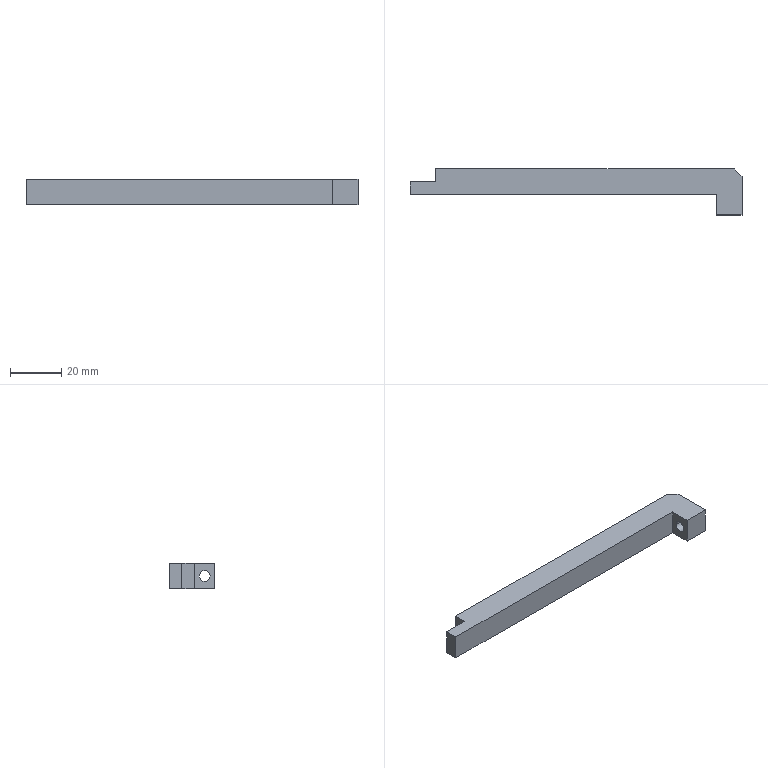Component | SolidWorks | SecondGenerationFour-sidedLabelingFeedingFrontLimitPlate-1 | 1 solid | 13 faces | box 130 x 18 x 10 mm | volume 13116 mm3 | plane 11 | cylinder 2 | commonest cylinder face diameters 4.2 x2
build123d program:
from build123d import *

# Parameters (mm, degrees)
SKETCH1_W             = 120
SKETCH1_H             = 10
BOSS_EXTRUDE1_DEPTH   = 10
SKETCH2_W             = 10
SKETCH2_H             = 10
BOSS_EXTRUDE2_DEPTH   = 8
M5_TAPPED_HOLE1_D     = 4.2
M5_TAPPED_HOLE1_DEPTH = 19
M5_TAPPED_HOLE1_TIP   = 1.262
SKETCH6_W             = 5
SKETCH6_H             = 10
BOSS_EXTRUDE4_DEPTH   = 10
CHAMFER1_SIZE         = 3


with BuildPart() as part:
    # Sketch1 → Boss-Extrude1 (new body)
    with BuildSketch(Plane.XY):
        with Locations((6.487, -24.142)):
            Rectangle(SKETCH1_W, SKETCH1_H)
    extrude(amount=BOSS_EXTRUDE1_DEPTH)

    # Sketch2 → Boss-Extrude2 (add)
    with BuildSketch(Plane(origin=(0, 0, 0), x_dir=(-1, 0, 0), z_dir=(0, 0, -1))):
        with Locations((-61.487, -24.142)):
            Rectangle(SKETCH2_W, SKETCH2_H)
    extrude(amount=BOSS_EXTRUDE2_DEPTH)

    # M5 Tapped Hole1
    with Locations(Plane(origin=(66.487, 0, 0), x_dir=(0, 0, -1), z_dir=(1, 0, 0))):
        with Locations((4, -24.142)):
            Hole(M5_TAPPED_HOLE1_D / 2, depth=M5_TAPPED_HOLE1_DEPTH)
            with Locations((0, 0, -(M5_TAPPED_HOLE1_DEPTH + M5_TAPPED_HOLE1_TIP / 2))):  # 118° drill point
                Cone(0, M5_TAPPED_HOLE1_D / 2, M5_TAPPED_HOLE1_TIP, mode=Mode.SUBTRACT)

    # Sketch6 → Boss-Extrude4 (add)
    with BuildSketch(Plane.ZY.offset(53.513)):
        with Locations((2.5, -24.142)):
            Rectangle(SKETCH6_W, SKETCH6_H)
    extrude(amount=BOSS_EXTRUDE4_DEPTH)

    # Chamfer1
    chamfer1_edges = [part.edges().sort_by_distance(p)[0] for p in [
        (66.487, -24.142, 10),
    ]]
    chamfer(chamfer1_edges, length=CHAMFER1_SIZE)


solid = part.part

# Placed as in the assembly
solid = solid.moved(Location((-16.514, 41.863, -216.142), (-90, 0, 0)))
STEP:
#1=COLOUR_RGB('',0.7922,0.8196,0.9333);
#2=FILL_AREA_STYLE_COLOUR('',#1);
#3=FILL_AREA_STYLE('',(#2));
#4=SURFACE_STYLE_FILL_AREA(#3);
#5=SURFACE_SIDE_STYLE('',(#4));
#6=SURFACE_STYLE_USAGE(.BOTH.,#5);
#7=PRESENTATION_STYLE_ASSIGNMENT((#6));
#8=CARTESIAN_POINT('',(1.574,1.573,-7.559));
#9=VERTEX_POINT('',#8);
#10=CARTESIAN_POINT('',(1.574,1.408,-7.559));
#11=VERTEX_POINT('',#10);
#12=CARTESIAN_POINT('',(1.574,1.491,-7.559));
#13=DIRECTION('',(1.,0.,0.));
#14=DIRECTION('',(0.,0.,-1.));
#15=AXIS2_PLACEMENT_3D('',#12,#13,#14);
#16=CIRCLE('',#15,0.08268);
#17=EDGE_CURVE('',#9,#11,#16,.T.);
#18=ORIENTED_EDGE('',*,*,#17,.F.);
#19=CARTESIAN_POINT('',(1.967,1.573,-7.559));
#20=VERTEX_POINT('',#19);
#21=CARTESIAN_POINT('',(1.967,1.573,-7.559));
#22=DIRECTION('',(1.,0.,0.));
#23=VECTOR('',#22,39.37);
#24=LINE('',#21,#23);
#25=EDGE_CURVE('',#9,#20,#24,.T.);
#26=ORIENTED_EDGE('',*,*,#25,.T.);
#27=CARTESIAN_POINT('',(1.967,1.408,-7.559));
#28=VERTEX_POINT('',#27);
#29=CARTESIAN_POINT('',(1.967,1.491,-7.559));
#30=DIRECTION('',(1.,0.,0.));
#31=DIRECTION('',(0.,-1.,0.));
#32=AXIS2_PLACEMENT_3D('',#29,#30,#31);
#33=CIRCLE('',#32,0.08268);
#34=EDGE_CURVE('',#20,#28,#33,.T.);
#35=ORIENTED_EDGE('',*,*,#34,.T.);
#36=CARTESIAN_POINT('',(1.967,1.408,-7.559));
#37=DIRECTION('',(1.,0.,0.));
#38=VECTOR('',#37,39.37);
#39=LINE('',#36,#38);
#40=EDGE_CURVE('',#11,#28,#39,.T.);
#41=ORIENTED_EDGE('',*,*,#40,.F.);
#42=EDGE_LOOP('',(#18,#26,#35,#41));
#43=FACE_OUTER_BOUND('',#42,.T.);
#44=CARTESIAN_POINT('',(1.967,1.491,-7.559));
#45=DIRECTION('',(1.,0.,0.));
#46=DIRECTION('',(0.,-1.,0.));
#47=AXIS2_PLACEMENT_3D('',#44,#45,#46);
#48=CYLINDRICAL_SURFACE('',#47,0.08268);
#49=ADVANCED_FACE('',(#43),#48,.F.);
#50=CARTESIAN_POINT('',(-2.757,1.845,-7.362));
#51=VERTEX_POINT('',#50);
#52=CARTESIAN_POINT('',(-2.757,1.845,-7.756));
#53=VERTEX_POINT('',#52);
#54=CARTESIAN_POINT('',(-2.757,1.845,-7.756));
#55=DIRECTION('',(0.,0.,-1.));
#56=VECTOR('',#55,39.37);
#57=LINE('',#54,#56);
#58=EDGE_CURVE('',#51,#53,#57,.T.);
#59=ORIENTED_EDGE('',*,*,#58,.F.);
#60=CARTESIAN_POINT('',(-2.757,2.042,-7.362));
#61=VERTEX_POINT('',#60);
#62=CARTESIAN_POINT('',(-2.757,2.042,-7.362));
#63=DIRECTION('',(0.,-1.,0.));
#64=VECTOR('',#63,39.37);
#65=LINE('',#62,#64);
#66=EDGE_CURVE('',#61,#51,#65,.T.);
#67=ORIENTED_EDGE('',*,*,#66,.F.);
#68=CARTESIAN_POINT('',(-2.757,2.042,-7.756));
#69=VERTEX_POINT('',#68);
#70=CARTESIAN_POINT('',(-2.757,2.042,-7.756));
#71=DIRECTION('',(0.,0.,1.));
#72=VECTOR('',#71,39.37);
#73=LINE('',#70,#72);
#74=EDGE_CURVE('',#69,#61,#73,.T.);
#75=ORIENTED_EDGE('',*,*,#74,.F.);
#76=CARTESIAN_POINT('',(-2.757,2.042,-7.756));
#77=DIRECTION('',(0.,-1.,0.));
#78=VECTOR('',#77,39.37);
#79=LINE('',#76,#78);
#80=EDGE_CURVE('',#69,#53,#79,.T.);
#81=ORIENTED_EDGE('',*,*,#80,.T.);
#82=EDGE_LOOP('',(#59,#67,#75,#81));
#83=FACE_OUTER_BOUND('',#82,.T.);
#84=CARTESIAN_POINT('',(-2.757,2.042,-7.756));
#85=DIRECTION('',(1.,0.,0.));
#86=DIRECTION('',(0.,-1.,0.));
#87=AXIS2_PLACEMENT_3D('',#84,#85,#86);
#88=PLANE('',#87);
#89=ADVANCED_FACE('',(#83),#88,.F.);
#90=CARTESIAN_POINT('',(1.574,1.648,-7.362));
#91=VERTEX_POINT('',#90);
#92=CARTESIAN_POINT('',(1.574,1.648,-7.756));
#93=VERTEX_POINT('',#92);
#94=CARTESIAN_POINT('',(1.574,1.648,-7.756));
#95=DIRECTION('',(0.,0.,-1.));
#96=VECTOR('',#95,39.37);
#97=LINE('',#94,#96);
#98=EDGE_CURVE('',#91,#93,#97,.T.);
#99=ORIENTED_EDGE('',*,*,#98,.F.);
#100=CARTESIAN_POINT('',(-3.151,1.648,-7.362));
#101=VERTEX_POINT('',#100);
#102=CARTESIAN_POINT('',(-2.757,1.648,-7.362));
#103=DIRECTION('',(1.,0.,0.));
#104=VECTOR('',#103,39.37);
#105=LINE('',#102,#104);
#106=EDGE_CURVE('',#101,#91,#105,.T.);
#107=ORIENTED_EDGE('',*,*,#106,.F.);
#108=CARTESIAN_POINT('',(-3.151,1.648,-7.756));
#109=VERTEX_POINT('',#108);
#110=CARTESIAN_POINT('',(-3.151,1.648,-7.756));
#111=DIRECTION('',(0.,0.,1.));
#112=VECTOR('',#111,39.37);
#113=LINE('',#110,#112);
#114=EDGE_CURVE('',#109,#101,#113,.T.);
#115=ORIENTED_EDGE('',*,*,#114,.F.);
#116=CARTESIAN_POINT('',(-2.757,1.648,-7.756));
#117=DIRECTION('',(-1.,0.,0.));
#118=VECTOR('',#117,39.37);
#119=LINE('',#116,#118);
#120=EDGE_CURVE('',#93,#109,#119,.T.);
#121=ORIENTED_EDGE('',*,*,#120,.F.);
#122=EDGE_LOOP('',(#99,#107,#115,#121));
#123=FACE_OUTER_BOUND('',#122,.T.);
#124=CARTESIAN_POINT('',(-2.757,1.648,-7.362));
#125=DIRECTION('',(0.,1.,0.));
#126=DIRECTION('',(1.,0.,0.));
#127=AXIS2_PLACEMENT_3D('',#124,#125,#126);
#128=PLANE('',#127);
#129=ADVANCED_FACE('',(#123),#128,.F.);
#130=CARTESIAN_POINT('',(1.967,1.924,-7.362));
#131=VERTEX_POINT('',#130);
#132=CARTESIAN_POINT('',(1.967,1.333,-7.362));
#133=VERTEX_POINT('',#132);
#134=CARTESIAN_POINT('',(1.967,2.042,-7.362));
#135=DIRECTION('',(0.,-1.,0.));
#136=VECTOR('',#135,39.37);
#137=LINE('',#134,#136);
#138=EDGE_CURVE('',#131,#133,#137,.T.);
#139=ORIENTED_EDGE('',*,*,#138,.F.);
#140=CARTESIAN_POINT('',(1.849,2.042,-7.362));
#141=VERTEX_POINT('',#140);
#142=CARTESIAN_POINT('',(1.849,2.042,-7.362));
#143=DIRECTION('',(-0.7071,0.7071,0.));
#144=VECTOR('',#143,39.37);
#145=LINE('',#142,#144);
#146=EDGE_CURVE('',#131,#141,#145,.T.);
#147=ORIENTED_EDGE('',*,*,#146,.T.);
#148=CARTESIAN_POINT('',(-2.757,2.042,-7.362));
#149=DIRECTION('',(1.,0.,0.));
#150=VECTOR('',#149,39.37);
#151=LINE('',#148,#150);
#152=EDGE_CURVE('',#61,#141,#151,.T.);
#153=ORIENTED_EDGE('',*,*,#152,.F.);
#154=ORIENTED_EDGE('',*,*,#66,.T.);
#155=CARTESIAN_POINT('',(-3.151,1.845,-7.362));
#156=VERTEX_POINT('',#155);
#157=CARTESIAN_POINT('',(-3.151,1.845,-7.362));
#158=DIRECTION('',(1.,0.,0.));
#159=VECTOR('',#158,39.37);
#160=LINE('',#157,#159);
#161=EDGE_CURVE('',#156,#51,#160,.T.);
#162=ORIENTED_EDGE('',*,*,#161,.F.);
#163=CARTESIAN_POINT('',(-3.151,1.648,-7.362));
#164=DIRECTION('',(0.,1.,0.));
#165=VECTOR('',#164,39.37);
#166=LINE('',#163,#165);
#167=EDGE_CURVE('',#101,#156,#166,.T.);
#168=ORIENTED_EDGE('',*,*,#167,.F.);
#169=ORIENTED_EDGE('',*,*,#106,.T.);
#170=CARTESIAN_POINT('',(1.574,1.333,-7.362));
#171=VERTEX_POINT('',#170);
#172=CARTESIAN_POINT('',(1.574,1.333,-7.362));
#173=DIRECTION('',(0.,1.,0.));
#174=VECTOR('',#173,39.37);
#175=LINE('',#172,#174);
#176=EDGE_CURVE('',#171,#91,#175,.T.);
#177=ORIENTED_EDGE('',*,*,#176,.F.);
#178=CARTESIAN_POINT('',(1.967,1.333,-7.362));
#179=DIRECTION('',(-1.,0.,0.));
#180=VECTOR('',#179,39.37);
#181=LINE('',#178,#180);
#182=EDGE_CURVE('',#133,#171,#181,.T.);
#183=ORIENTED_EDGE('',*,*,#182,.F.);
#184=EDGE_LOOP('',(#139,#147,#153,#154,#162,#168,#169,#177,#183));
#185=FACE_OUTER_BOUND('',#184,.T.);
#186=CARTESIAN_POINT('',(-2.757,2.042,-7.362));
#187=DIRECTION('',(0.,0.,-1.));
#188=DIRECTION('',(0.,1.,0.));
#189=AXIS2_PLACEMENT_3D('',#186,#187,#188);
#190=PLANE('',#189);
#191=ADVANCED_FACE('',(#185),#190,.F.);
#192=CARTESIAN_POINT('',(1.967,1.491,-7.559));
#193=DIRECTION('',(1.,0.,0.));
#194=DIRECTION('',(0.,-1.,0.));
#195=AXIS2_PLACEMENT_3D('',#192,#193,#194);
#196=CIRCLE('',#195,0.08268);
#197=EDGE_CURVE('',#28,#20,#196,.T.);
#198=ORIENTED_EDGE('',*,*,#197,.F.);
#199=ORIENTED_EDGE('',*,*,#34,.F.);
#200=EDGE_LOOP('',(#198,#199));
#201=FACE_BOUND('',#200,.T.);
#202=CARTESIAN_POINT('',(1.967,1.924,-7.756));
#203=VERTEX_POINT('',#202);
#204=CARTESIAN_POINT('',(1.967,1.333,-7.756));
#205=VERTEX_POINT('',#204);
#206=CARTESIAN_POINT('',(1.967,2.042,-7.756));
#207=DIRECTION('',(0.,-1.,0.));
#208=VECTOR('',#207,39.37);
#209=LINE('',#206,#208);
#210=EDGE_CURVE('',#203,#205,#209,.T.);
#211=ORIENTED_EDGE('',*,*,#210,.F.);
#212=CARTESIAN_POINT('',(1.967,1.924,-7.362));
#213=DIRECTION('',(0.,0.,1.));
#214=VECTOR('',#213,39.37);
#215=LINE('',#212,#214);
#216=EDGE_CURVE('',#203,#131,#215,.T.);
#217=ORIENTED_EDGE('',*,*,#216,.T.);
#218=ORIENTED_EDGE('',*,*,#138,.T.);
#219=CARTESIAN_POINT('',(1.967,1.333,-7.756));
#220=DIRECTION('',(0.,0.,1.));
#221=VECTOR('',#220,39.37);
#222=LINE('',#219,#221);
#223=EDGE_CURVE('',#205,#133,#222,.T.);
#224=ORIENTED_EDGE('',*,*,#223,.F.);
#225=EDGE_LOOP('',(#211,#217,#218,#224));
#226=FACE_OUTER_BOUND('',#225,.T.);
#227=CARTESIAN_POINT('',(1.967,2.042,-7.756));
#228=DIRECTION('',(-1.,0.,0.));
#229=DIRECTION('',(0.,1.,0.));
#230=AXIS2_PLACEMENT_3D('',#227,#228,#229);
#231=PLANE('',#230);
#232=ADVANCED_FACE('',(#201,#226),#231,.F.);
#233=CARTESIAN_POINT('',(1.849,2.042,-7.756));
#234=VERTEX_POINT('',#233);
#235=CARTESIAN_POINT('',(-2.757,2.042,-7.756));
#236=DIRECTION('',(-1.,0.,0.));
#237=VECTOR('',#236,39.37);
#238=LINE('',#235,#237);
#239=EDGE_CURVE('',#234,#69,#238,.T.);
#240=ORIENTED_EDGE('',*,*,#239,.F.);
#241=CARTESIAN_POINT('',(1.849,2.042,-7.756));
#242=DIRECTION('',(0.7071,-0.7071,0.));
#243=VECTOR('',#242,39.37);
#244=LINE('',#241,#243);
#245=EDGE_CURVE('',#234,#203,#244,.T.);
#246=ORIENTED_EDGE('',*,*,#245,.T.);
#247=ORIENTED_EDGE('',*,*,#210,.T.);
#248=CARTESIAN_POINT('',(1.574,1.333,-7.756));
#249=VERTEX_POINT('',#248);
#250=CARTESIAN_POINT('',(1.967,1.333,-7.756));
#251=DIRECTION('',(1.,0.,0.));
#252=VECTOR('',#251,39.37);
#253=LINE('',#250,#252);
#254=EDGE_CURVE('',#249,#205,#253,.T.);
#255=ORIENTED_EDGE('',*,*,#254,.F.);
#256=CARTESIAN_POINT('',(1.574,1.333,-7.756));
#257=DIRECTION('',(0.,1.,0.));
#258=VECTOR('',#257,39.37);
#259=LINE('',#256,#258);
#260=EDGE_CURVE('',#249,#93,#259,.T.);
#261=ORIENTED_EDGE('',*,*,#260,.T.);
#262=ORIENTED_EDGE('',*,*,#120,.T.);
#263=CARTESIAN_POINT('',(-3.151,1.845,-7.756));
#264=VERTEX_POINT('',#263);
#265=CARTESIAN_POINT('',(-3.151,1.648,-7.756));
#266=DIRECTION('',(0.,-1.,0.));
#267=VECTOR('',#266,39.37);
#268=LINE('',#265,#267);
#269=EDGE_CURVE('',#264,#109,#268,.T.);
#270=ORIENTED_EDGE('',*,*,#269,.F.);
#271=CARTESIAN_POINT('',(-3.151,1.845,-7.756));
#272=DIRECTION('',(1.,0.,0.));
#273=VECTOR('',#272,39.37);
#274=LINE('',#271,#273);
#275=EDGE_CURVE('',#264,#53,#274,.T.);
#276=ORIENTED_EDGE('',*,*,#275,.T.);
#277=ORIENTED_EDGE('',*,*,#80,.F.);
#278=EDGE_LOOP('',(#240,#246,#247,#255,#261,#262,#270,#276,#277));
#279=FACE_OUTER_BOUND('',#278,.T.);
#280=CARTESIAN_POINT('',(-2.757,2.042,-7.756));
#281=DIRECTION('',(0.,0.,1.));
#282=DIRECTION('',(0.,-1.,0.));
#283=AXIS2_PLACEMENT_3D('',#280,#281,#282);
#284=PLANE('',#283);
#285=ADVANCED_FACE('',(#279),#284,.F.);
#286=ORIENTED_EDGE('',*,*,#152,.T.);
#287=CARTESIAN_POINT('',(1.849,2.042,-7.756));
#288=DIRECTION('',(0.,0.,-1.));
#289=VECTOR('',#288,39.37);
#290=LINE('',#287,#289);
#291=EDGE_CURVE('',#141,#234,#290,.T.);
#292=ORIENTED_EDGE('',*,*,#291,.T.);
#293=ORIENTED_EDGE('',*,*,#239,.T.);
#294=ORIENTED_EDGE('',*,*,#74,.T.);
#295=EDGE_LOOP('',(#286,#292,#293,#294));
#296=FACE_OUTER_BOUND('',#295,.T.);
#297=CARTESIAN_POINT('',(-2.757,2.042,-7.362));
#298=DIRECTION('',(0.,1.,0.));
#299=DIRECTION('',(1.,0.,0.));
#300=AXIS2_PLACEMENT_3D('',#297,#298,#299);
#301=PLANE('',#300);
#302=ADVANCED_FACE('',(#296),#301,.T.);
#303=CARTESIAN_POINT('',(1.574,1.491,-7.559));
#304=DIRECTION('',(1.,0.,0.));
#305=DIRECTION('',(0.,0.,-1.));
#306=AXIS2_PLACEMENT_3D('',#303,#304,#305);
#307=CIRCLE('',#306,0.08268);
#308=EDGE_CURVE('',#11,#9,#307,.T.);
#309=ORIENTED_EDGE('',*,*,#308,.T.);
#310=ORIENTED_EDGE('',*,*,#17,.T.);
#311=EDGE_LOOP('',(#309,#310));
#312=FACE_BOUND('',#311,.T.);
#313=ORIENTED_EDGE('',*,*,#98,.T.);
#314=ORIENTED_EDGE('',*,*,#260,.F.);
#315=CARTESIAN_POINT('',(1.574,1.333,-7.756));
#316=DIRECTION('',(0.,0.,-1.));
#317=VECTOR('',#316,39.37);
#318=LINE('',#315,#317);
#319=EDGE_CURVE('',#171,#249,#318,.T.);
#320=ORIENTED_EDGE('',*,*,#319,.F.);
#321=ORIENTED_EDGE('',*,*,#176,.T.);
#322=EDGE_LOOP('',(#313,#314,#320,#321));
#323=FACE_OUTER_BOUND('',#322,.T.);
#324=CARTESIAN_POINT('',(1.574,1.333,-7.756));
#325=DIRECTION('',(1.,0.,0.));
#326=DIRECTION('',(0.,0.,-1.));
#327=AXIS2_PLACEMENT_3D('',#324,#325,#326);
#328=PLANE('',#327);
#329=ADVANCED_FACE('',(#312,#323),#328,.F.);
#330=ORIENTED_EDGE('',*,*,#223,.T.);
#331=ORIENTED_EDGE('',*,*,#182,.T.);
#332=ORIENTED_EDGE('',*,*,#319,.T.);
#333=ORIENTED_EDGE('',*,*,#254,.T.);
#334=EDGE_LOOP('',(#330,#331,#332,#333));
#335=FACE_OUTER_BOUND('',#334,.T.);
#336=CARTESIAN_POINT('',(1.967,1.333,-7.362));
#337=DIRECTION('',(0.,-1.,0.));
#338=DIRECTION('',(-1.,0.,0.));
#339=AXIS2_PLACEMENT_3D('',#336,#337,#338);
#340=PLANE('',#339);
#341=ADVANCED_FACE('',(#335),#340,.T.);
#342=ORIENTED_EDGE('',*,*,#25,.F.);
#343=ORIENTED_EDGE('',*,*,#308,.F.);
#344=ORIENTED_EDGE('',*,*,#40,.T.);
#345=ORIENTED_EDGE('',*,*,#197,.T.);
#346=EDGE_LOOP('',(#342,#343,#344,#345));
#347=FACE_OUTER_BOUND('',#346,.T.);
#348=CARTESIAN_POINT('',(1.967,1.491,-7.559));
#349=DIRECTION('',(1.,0.,0.));
#350=DIRECTION('',(0.,-1.,0.));
#351=AXIS2_PLACEMENT_3D('',#348,#349,#350);
#352=CYLINDRICAL_SURFACE('',#351,0.08268);
#353=ADVANCED_FACE('',(#347),#352,.F.);
#354=ORIENTED_EDGE('',*,*,#58,.T.);
#355=ORIENTED_EDGE('',*,*,#275,.F.);
#356=CARTESIAN_POINT('',(-3.151,1.845,-7.756));
#357=DIRECTION('',(0.,0.,-1.));
#358=VECTOR('',#357,39.37);
#359=LINE('',#356,#358);
#360=EDGE_CURVE('',#156,#264,#359,.T.);
#361=ORIENTED_EDGE('',*,*,#360,.F.);
#362=ORIENTED_EDGE('',*,*,#161,.T.);
#363=EDGE_LOOP('',(#354,#355,#361,#362));
#364=FACE_OUTER_BOUND('',#363,.T.);
#365=CARTESIAN_POINT('',(-3.151,1.845,-7.756));
#366=DIRECTION('',(0.,-1.,-0.));
#367=DIRECTION('',(0.,0.,-1.));
#368=AXIS2_PLACEMENT_3D('',#365,#366,#367);
#369=PLANE('',#368);
#370=ADVANCED_FACE('',(#364),#369,.F.);
#371=ORIENTED_EDGE('',*,*,#114,.T.);
#372=ORIENTED_EDGE('',*,*,#167,.T.);
#373=ORIENTED_EDGE('',*,*,#360,.T.);
#374=ORIENTED_EDGE('',*,*,#269,.T.);
#375=EDGE_LOOP('',(#371,#372,#373,#374));
#376=FACE_OUTER_BOUND('',#375,.T.);
#377=CARTESIAN_POINT('',(-3.151,1.648,-7.362));
#378=DIRECTION('',(-1.,0.,0.));
#379=DIRECTION('',(0.,1.,0.));
#380=AXIS2_PLACEMENT_3D('',#377,#378,#379);
#381=PLANE('',#380);
#382=ADVANCED_FACE('',(#376),#381,.T.);
#383=ORIENTED_EDGE('',*,*,#146,.F.);
#384=ORIENTED_EDGE('',*,*,#216,.F.);
#385=ORIENTED_EDGE('',*,*,#245,.F.);
#386=ORIENTED_EDGE('',*,*,#291,.F.);
#387=EDGE_LOOP('',(#383,#384,#385,#386));
#388=FACE_OUTER_BOUND('',#387,.T.);
#389=CARTESIAN_POINT('',(1.849,2.042,-7.362));
#390=DIRECTION('',(0.7071,0.7071,0.));
#391=DIRECTION('',(0.,0.,1.));
#392=AXIS2_PLACEMENT_3D('',#389,#390,#391);
#393=PLANE('',#392);
#394=ADVANCED_FACE('',(#388),#393,.T.);
#395=CLOSED_SHELL('',(#49,#89,#129,#191,#232,#285,#302,#329,#341,#353,#370,#382,#394));
#396=MANIFOLD_SOLID_BREP('',#395);
#397=STYLED_ITEM('',(#7),#396);
#398=PRESENTATION_LAYER_ASSIGNMENT('','',(#397));
#399=CARTESIAN_POINT('',(0.,0.,0.));
#400=DIRECTION('',(0.,0.,1.));
#401=DIRECTION('',(1.,0.,0.));
#402=AXIS2_PLACEMENT_3D('',#399,#400,#401);
#403=(LENGTH_UNIT()NAMED_UNIT(*)SI_UNIT($,.METRE.));
#404=LENGTH_MEASURE_WITH_UNIT(LENGTH_MEASURE(0.0254),#403);
#405=DIMENSIONAL_EXPONENTS(1.,0.,0.,0.,0.,0.,0.);
#406=(CONVERSION_BASED_UNIT('',#404)LENGTH_UNIT()NAMED_UNIT(#405));
#407=UNCERTAINTY_MEASURE_WITH_UNIT(LENGTH_MEASURE(0.00001),#406,'','');
#408=(NAMED_UNIT(*)PLANE_ANGLE_UNIT()SI_UNIT($,.RADIAN.));
#409=(NAMED_UNIT(*)SI_UNIT($,.STERADIAN.)SOLID_ANGLE_UNIT());
#410=(GEOMETRIC_REPRESENTATION_CONTEXT(3)GLOBAL_UNCERTAINTY_ASSIGNED_CONTEXT((#407))GLOBAL_UNIT_ASSIGNED_CONTEXT((#406,#408,#409))REPRESENTATION_CONTEXT('',''));
#411=ADVANCED_BREP_SHAPE_REPRESENTATION('',(#396,#402),#410);
#412=(LENGTH_UNIT()NAMED_UNIT(*)SI_UNIT($,.METRE.));
#413=LENGTH_MEASURE_WITH_UNIT(LENGTH_MEASURE(0.0254),#412);
#414=DIMENSIONAL_EXPONENTS(1.,0.,0.,0.,0.,0.,0.);
#415=(CONVERSION_BASED_UNIT('',#413)LENGTH_UNIT()NAMED_UNIT(#414));
#416=UNCERTAINTY_MEASURE_WITH_UNIT(LENGTH_MEASURE(0.00001),#415,'','');
#417=(NAMED_UNIT(*)PLANE_ANGLE_UNIT()SI_UNIT($,.RADIAN.));
#418=(NAMED_UNIT(*)SI_UNIT($,.STERADIAN.)SOLID_ANGLE_UNIT());
#419=(GEOMETRIC_REPRESENTATION_CONTEXT(3)GLOBAL_UNCERTAINTY_ASSIGNED_CONTEXT((#416))GLOBAL_UNIT_ASSIGNED_CONTEXT((#415,#417,#418))REPRESENTATION_CONTEXT('',''));
#420=MECHANICAL_DESIGN_GEOMETRIC_PRESENTATION_REPRESENTATION('',(#397),#419);